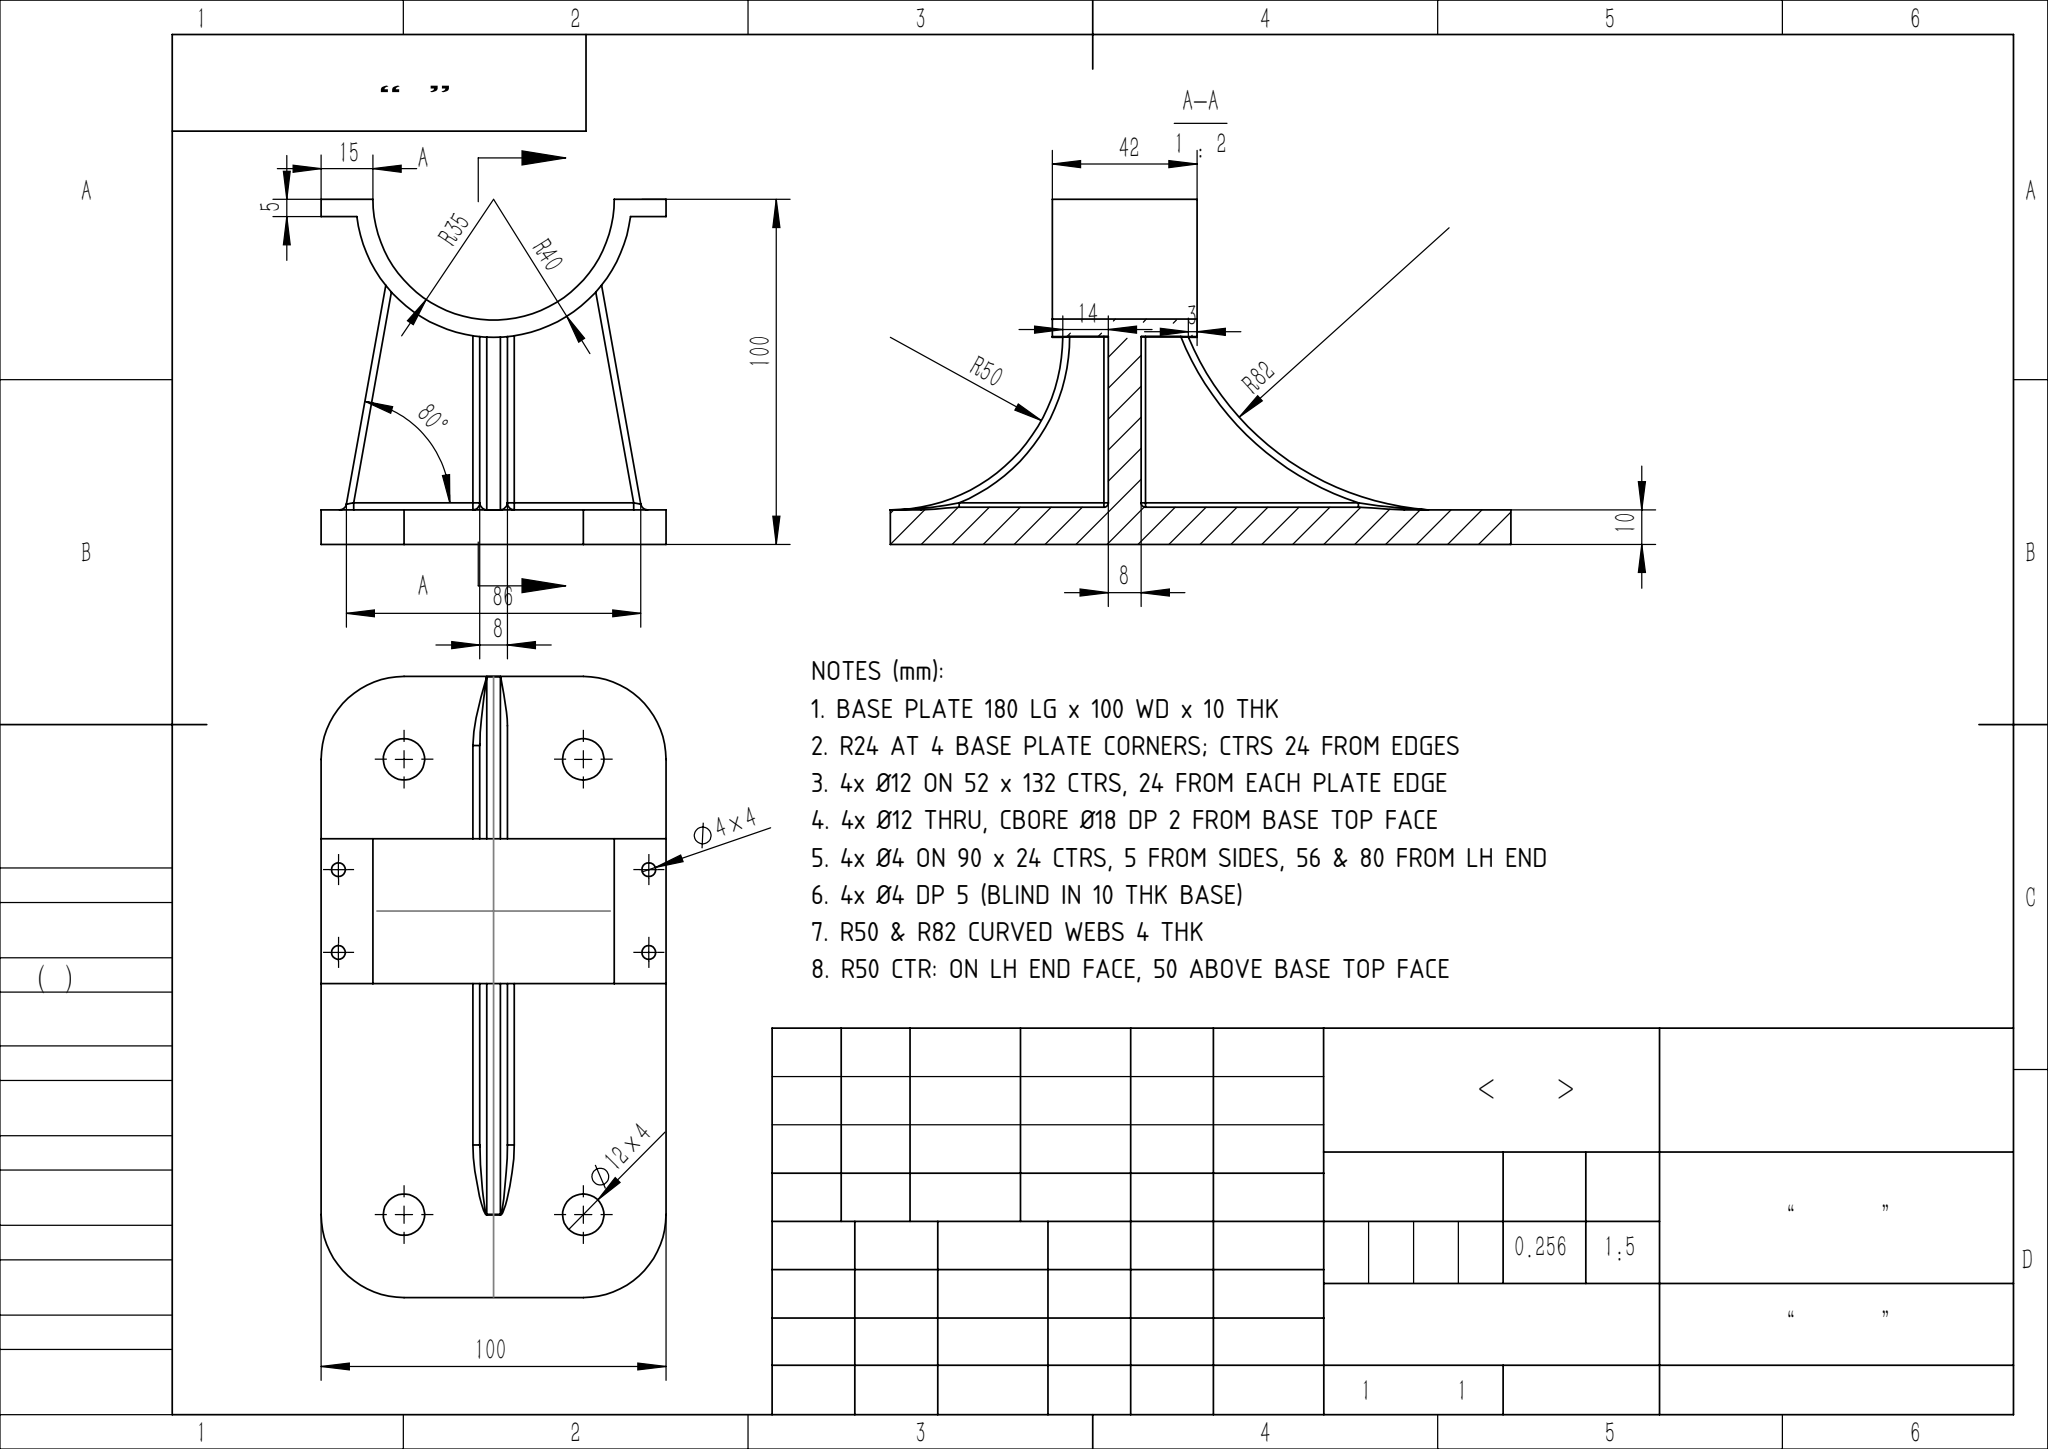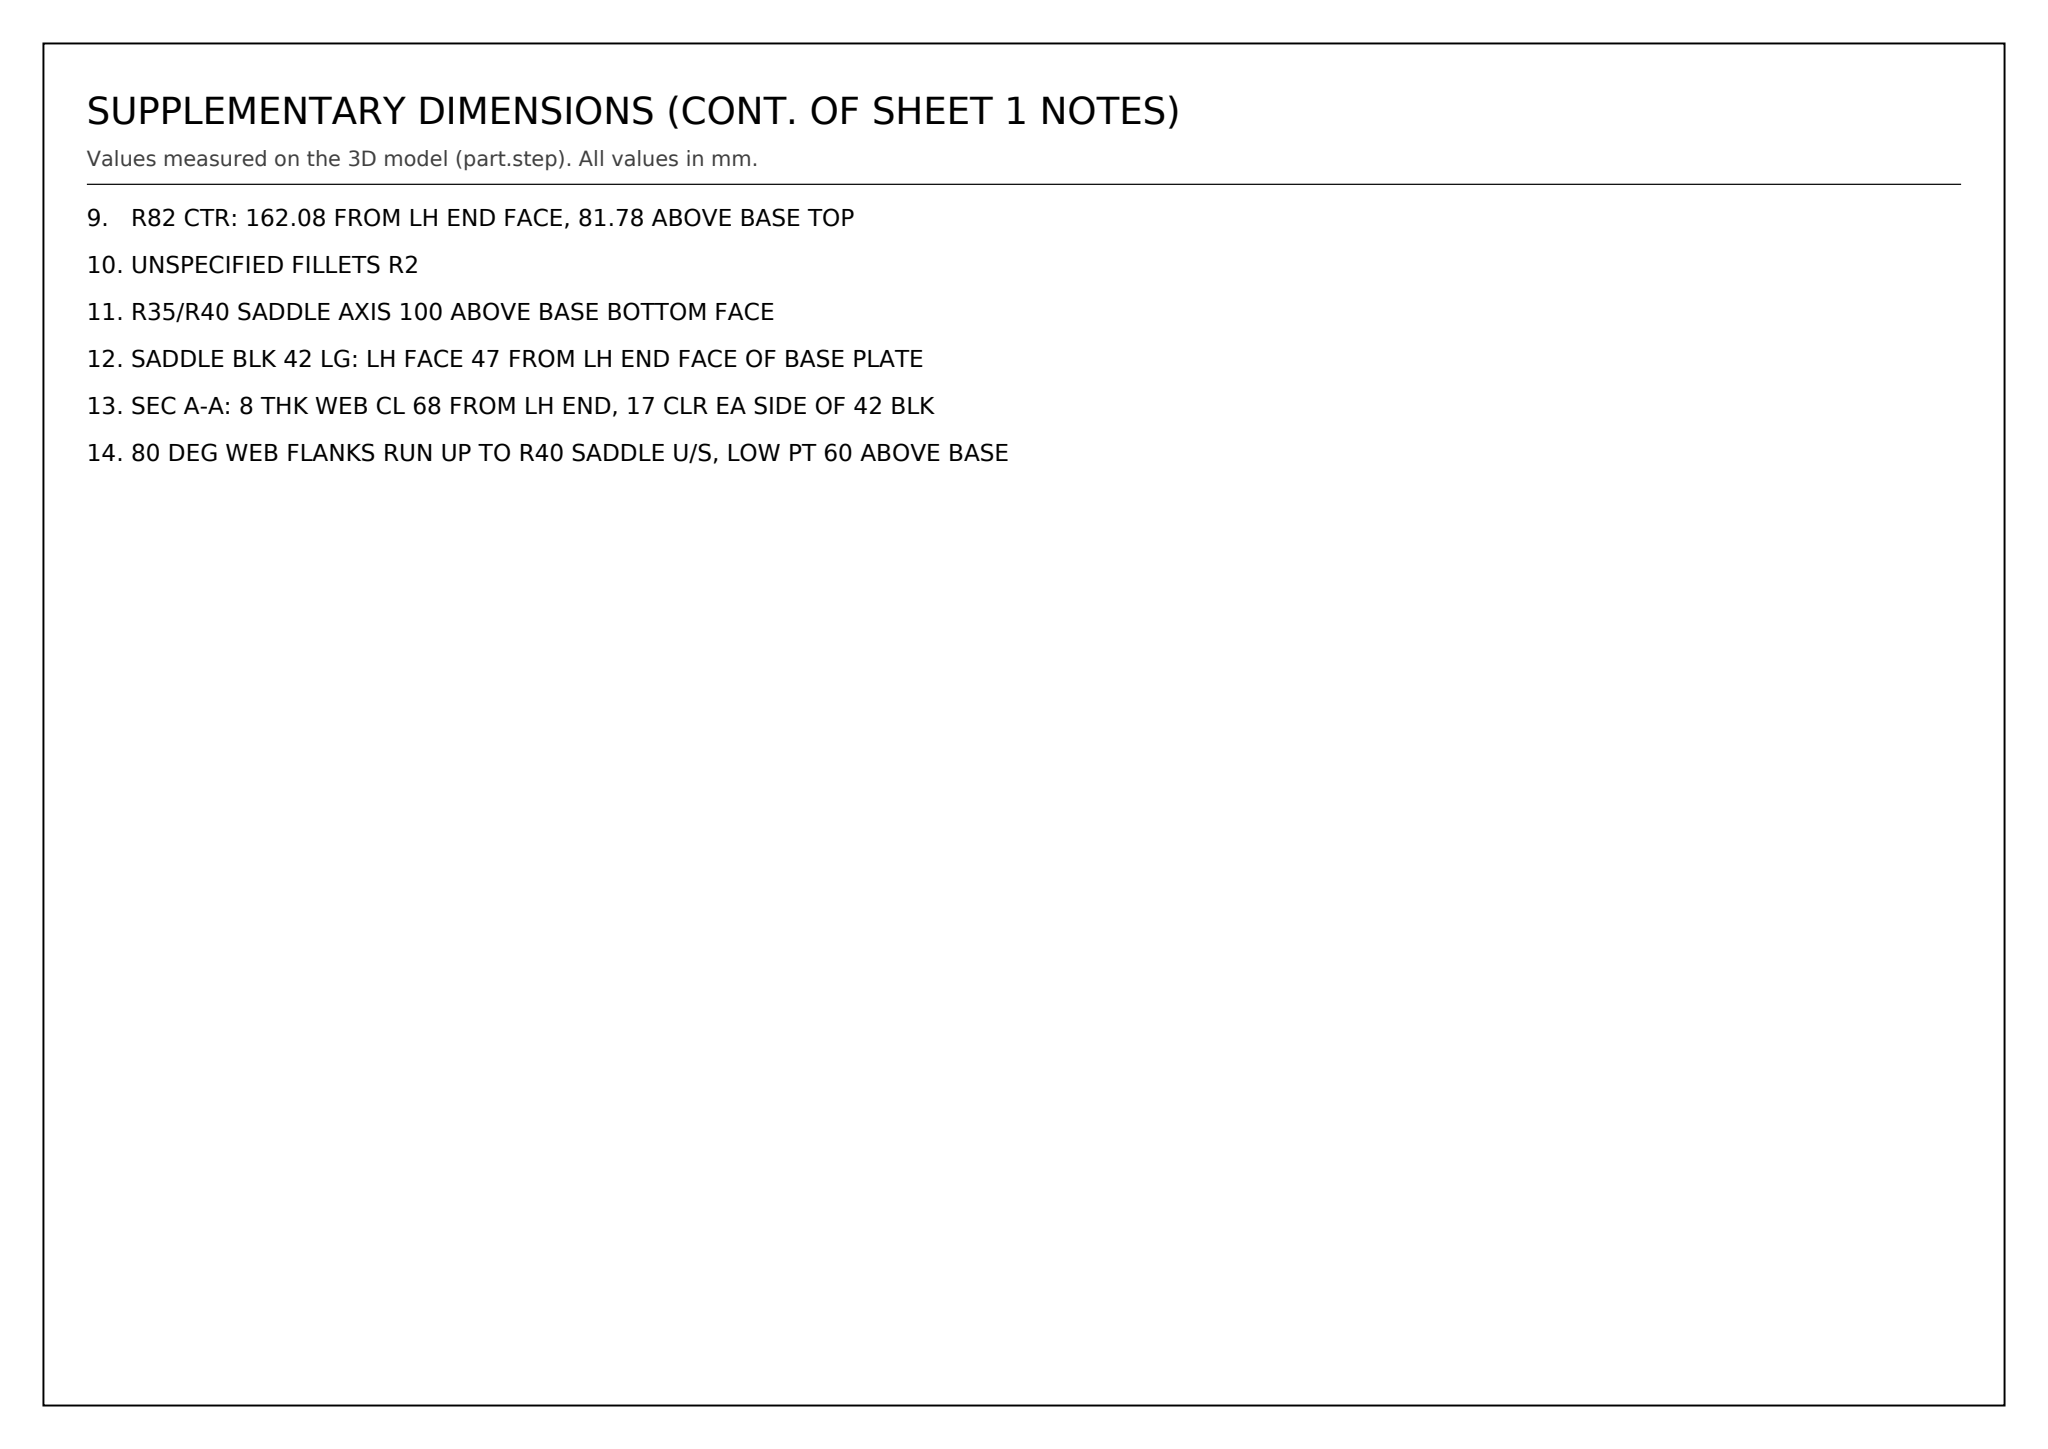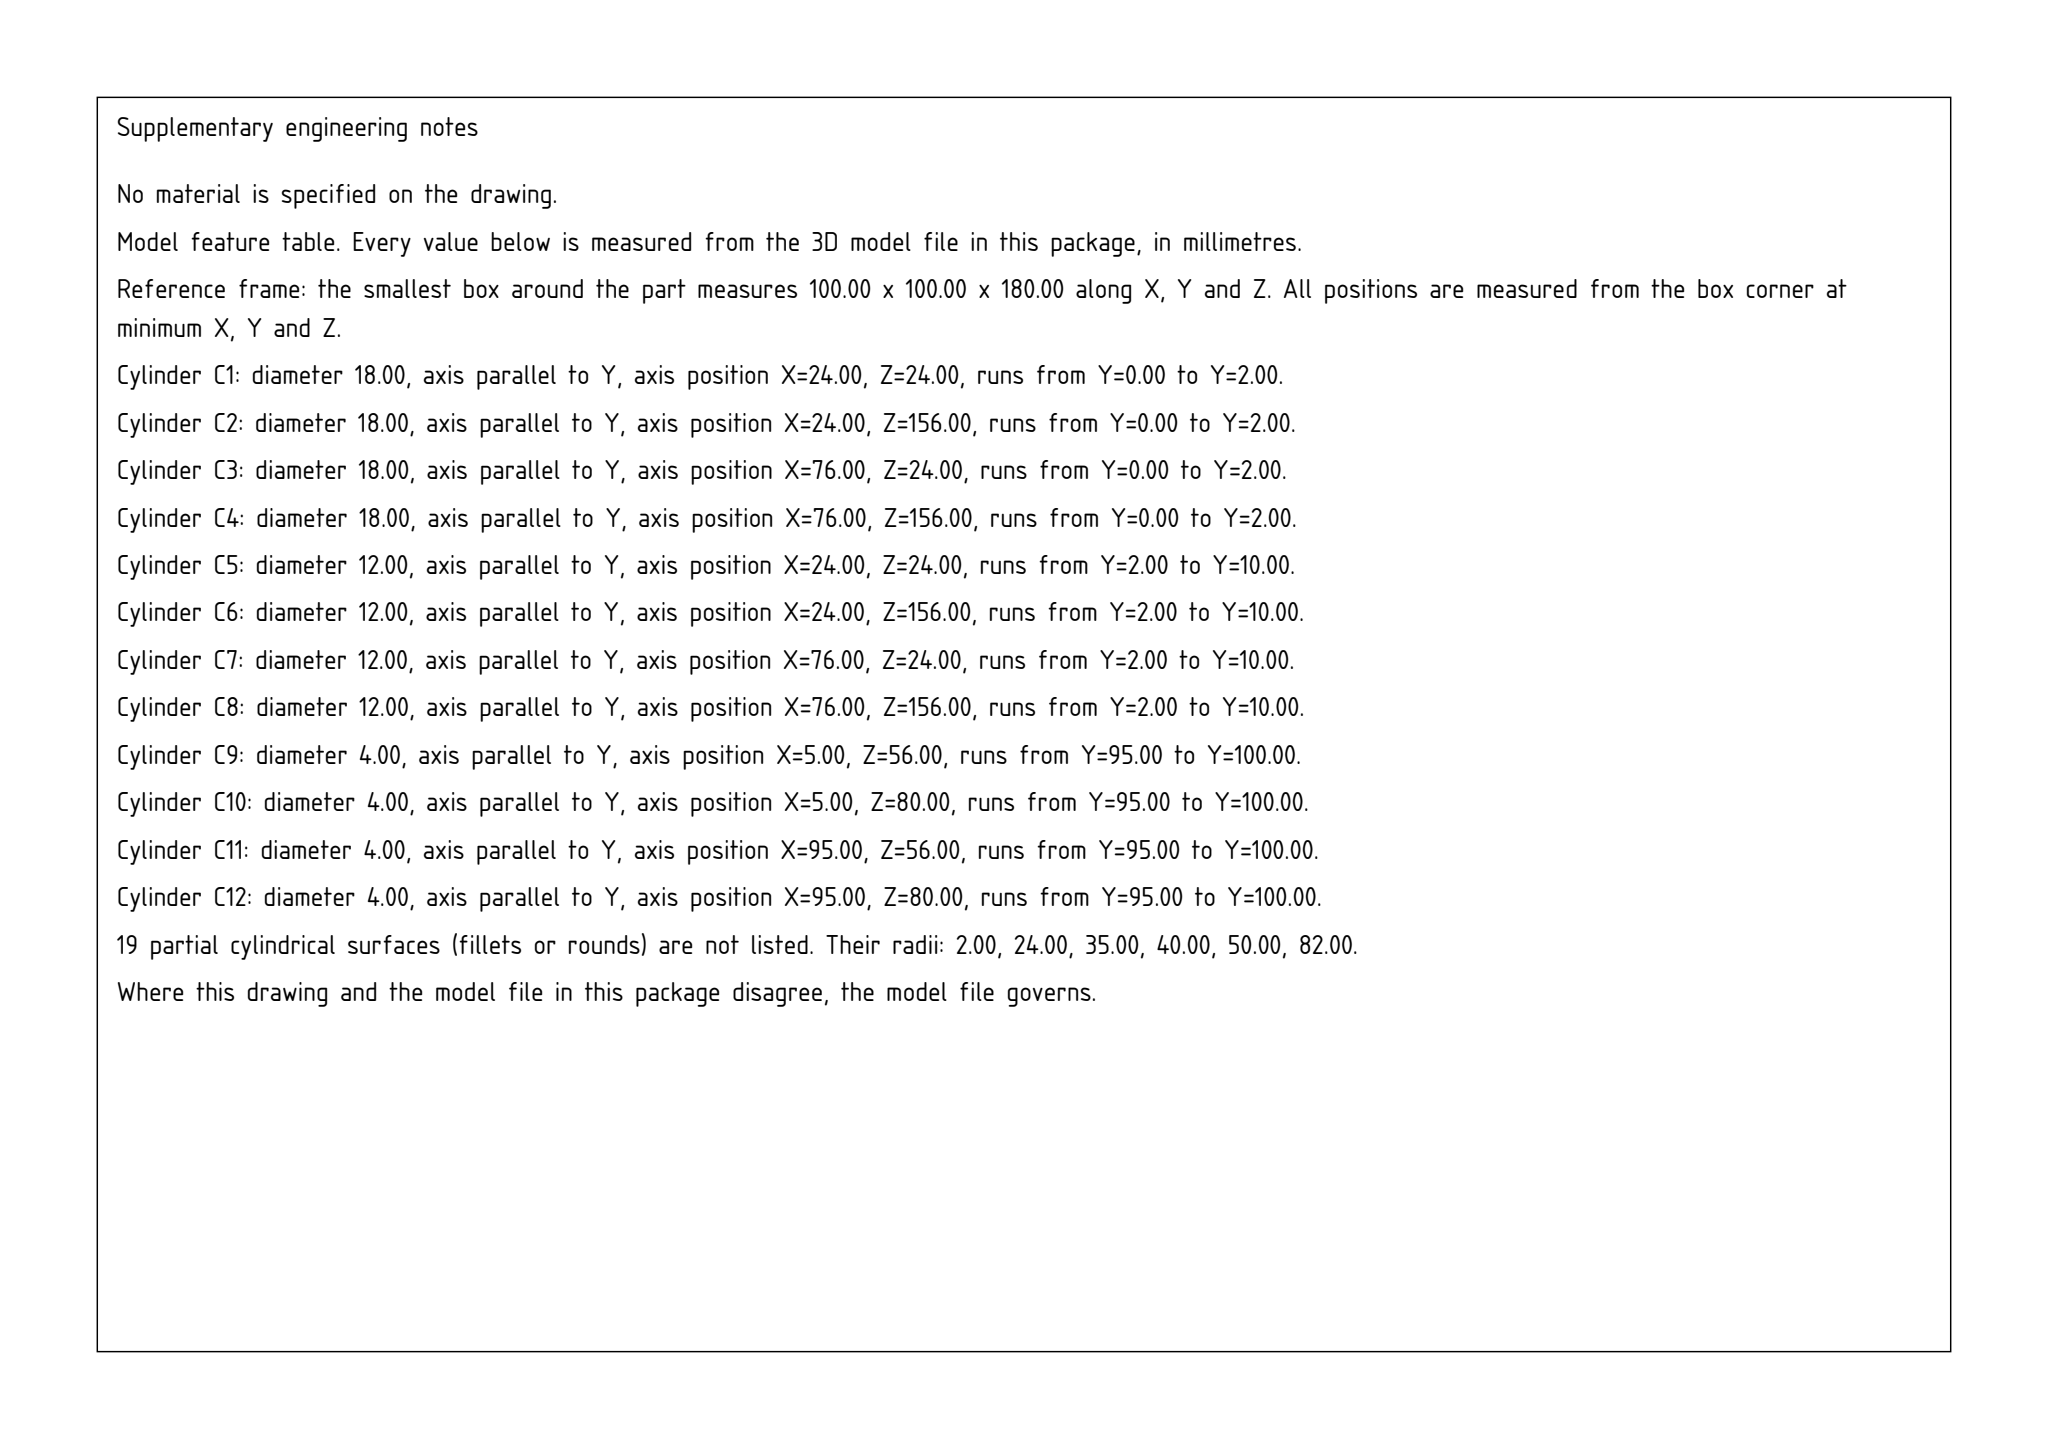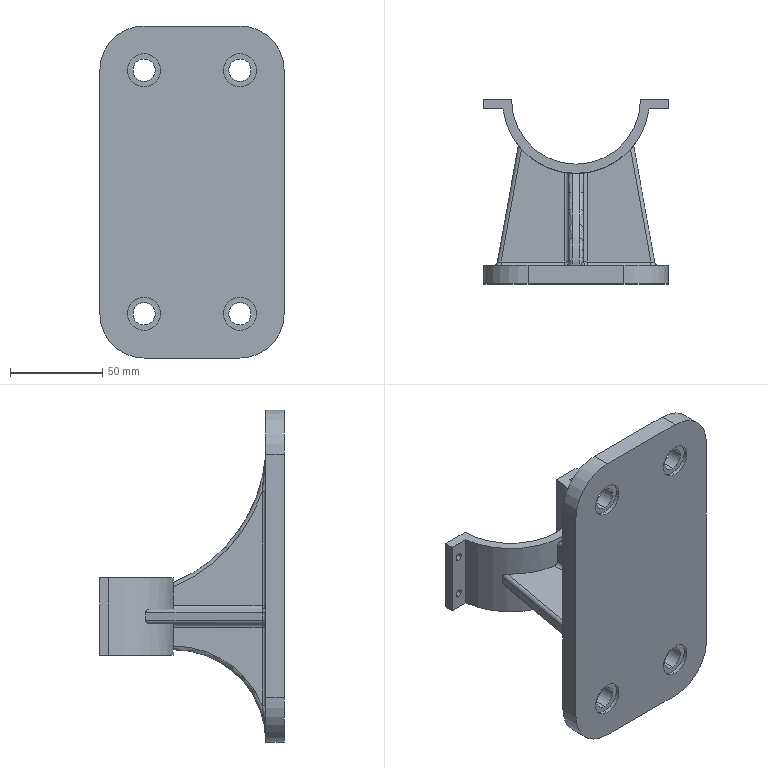Part | SolidWorks | mm | 1 solid | 94 faces | box 100 x 100 x 180 mm | volume 255527 mm3 | cylinder 50 | plane 28 | spline 7 | torus 6 | sphere 3 | commonest cylinder face diameters 4 x26 12 x8 18 x8 48 x4 80 x1 70 x1 100 x1 164 x1
Drawing notes:
BASE PLATE 180 LG x 100 WD x 10 THK | from the solid: bbox_xyz [100.001,100.424,180.001]; base y-planes 0.42 & 10.42 = 10 thk
R24 AT 4 BASE PLATE CORNERS; CTRS 24 FROM EDGES | from the solid: 4x Ø48 y-axis cyl, L=10, at (24,24),(24,156),(76,24),(76,156)
4x Ø12 ON 52 x 132 CTRS, 24 FROM EACH PLATE EDGE | from the solid: Ø12 y-axis holes at x=24/76, z=24/156; 76-24=52, 156-24=132
4x Ø12 THRU, CBORE Ø18 DP 2 FROM BASE TOP FACE | from the solid: Ø12 L=8 + Ø18 L=2 = 10 plate thk, same axes (24/76, 24/156)
4x Ø4 ON 90 x 24 CTRS, 5 FROM SIDES, 56 & 80 FROM LH END | from the solid: Ø4 y-axis holes at x=5 & 95, z=56 & 80 (95-5=90, 80-56=24)
4x Ø4 DP 5 (BLIND IN 10 THK BASE) | from the solid: Ø4 y-axis cyl length 5.0 at (5,56),(5,80),(95,56),(95,80)
R50 & R82 CURVED WEBS 4 THK | from the solid: Ø100 x-axis cyl L=4 (R50) and Ø164 x-axis cyl L=4 (R82)
R50 CTR: ON LH END FACE, 50 ABOVE BASE TOP FACE | from the solid: Ø100 x-axis cyl ctr at y=60.42, z=0.01; 60.42-10.42=50
R82 CTR: 162.08 FROM LH END FACE, 81.78 ABOVE BASE TOP | from the solid: Ø164 x-axis cyl ctr at y=92.2, z=162.08; 92.2-10.42=81.78
UNSPECIFIED FILLETS R2 | from the solid: fillet_radii [[2.0,6]] - six R2 fillets at web/rib/base joins
R35/R40 SADDLE AXIS 100 ABOVE BASE BOTTOM FACE | from the solid: Ø70/Ø80 z-axis cyl axis at y=100.42; base btm y=0.42 -> 100
SADDLE BLK 42 LG: LH FACE 47 FROM LH END FACE OF BASE PLATE | from the solid: z-planes 47 and 89 (42 apart) bound the D80/D70 saddle; base plate z=0..180
SEC A-A: 8 THK WEB CL 68 FROM LH END, 17 CLR EA SIDE OF 42 BLK | from the solid: z-planes 64 & 72 (8 thk), CL z=68; 64-47=17 and 89-72=17
80 DEG WEB FLANKS RUN UP TO R40 SADDLE U/S, LOW PT 60 ABOVE BASE | from the solid: D80 cyl axis y=100.42, R40 -> u/s low pt y=60.42; base underside y=0.42